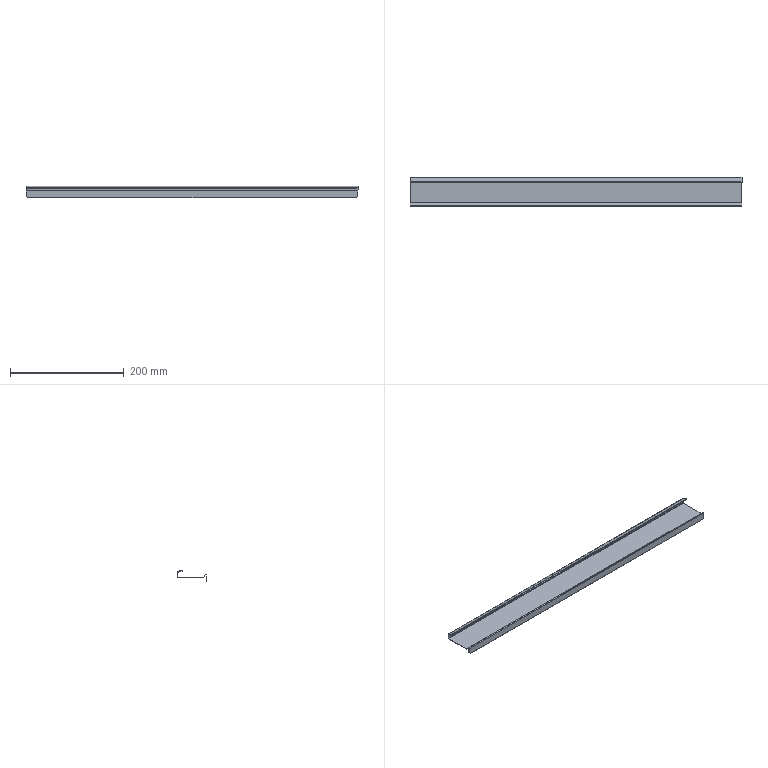Component | SolidWorks | PC-CAJ-P08-1_PC-CAJ-P16-1_PM-CAJ-P51-1 | 1 solid | 50 faces | volume 38008 mm3 | plane 38 | cylinder 12 | commonest cylinder face diameters 2.4 x5 1 x4 0.2 x2 1.6 x1 | material Plain Carbon Steel